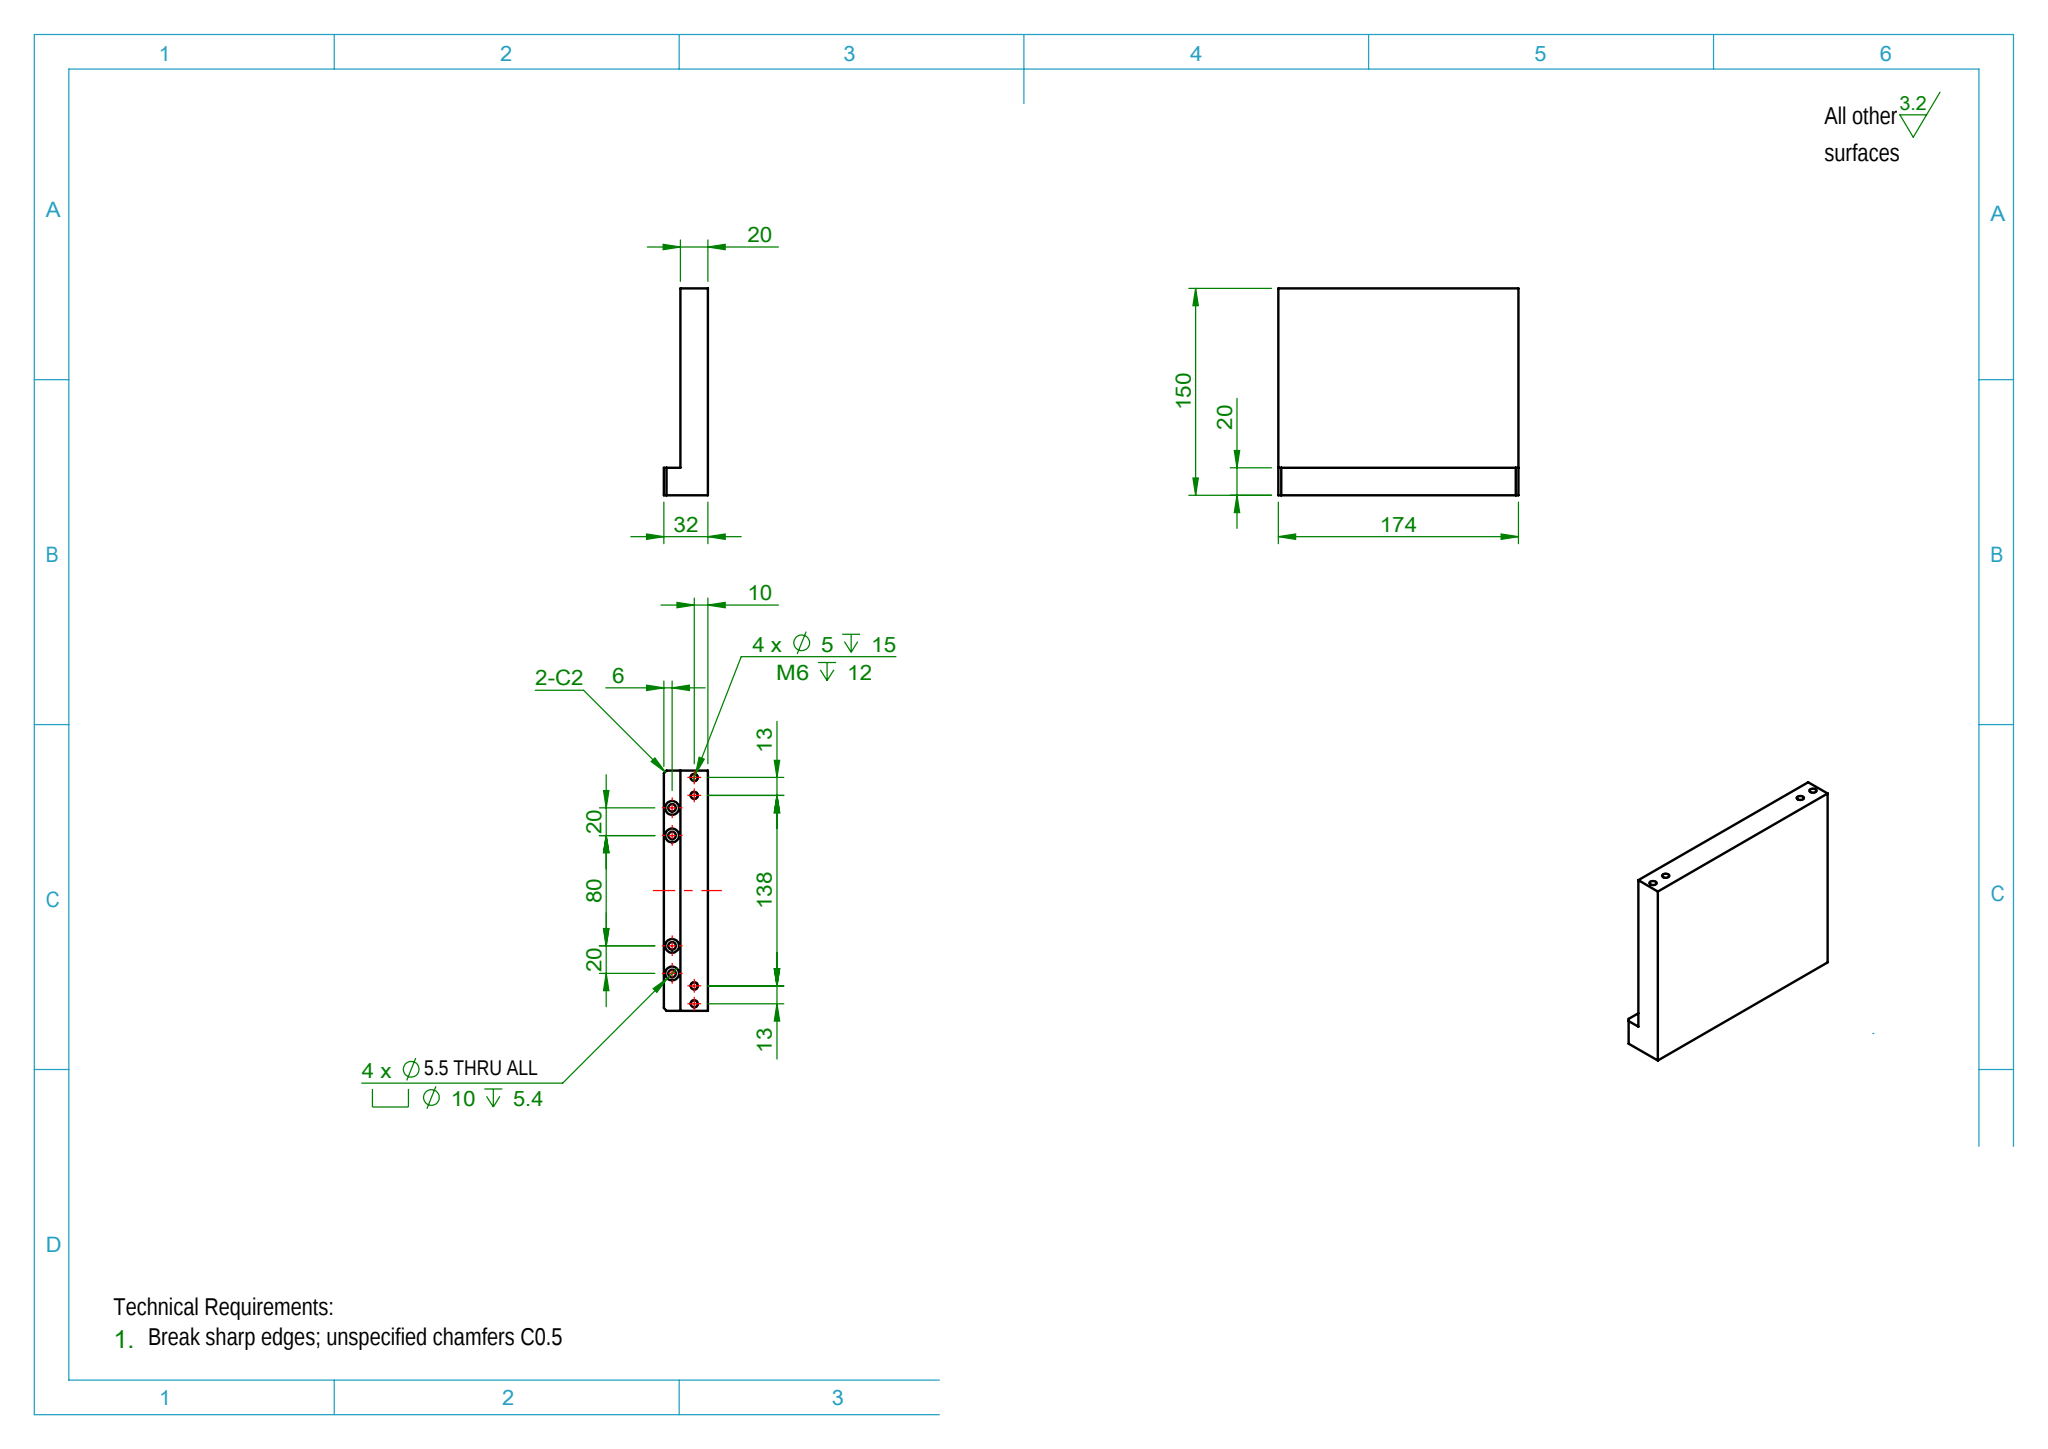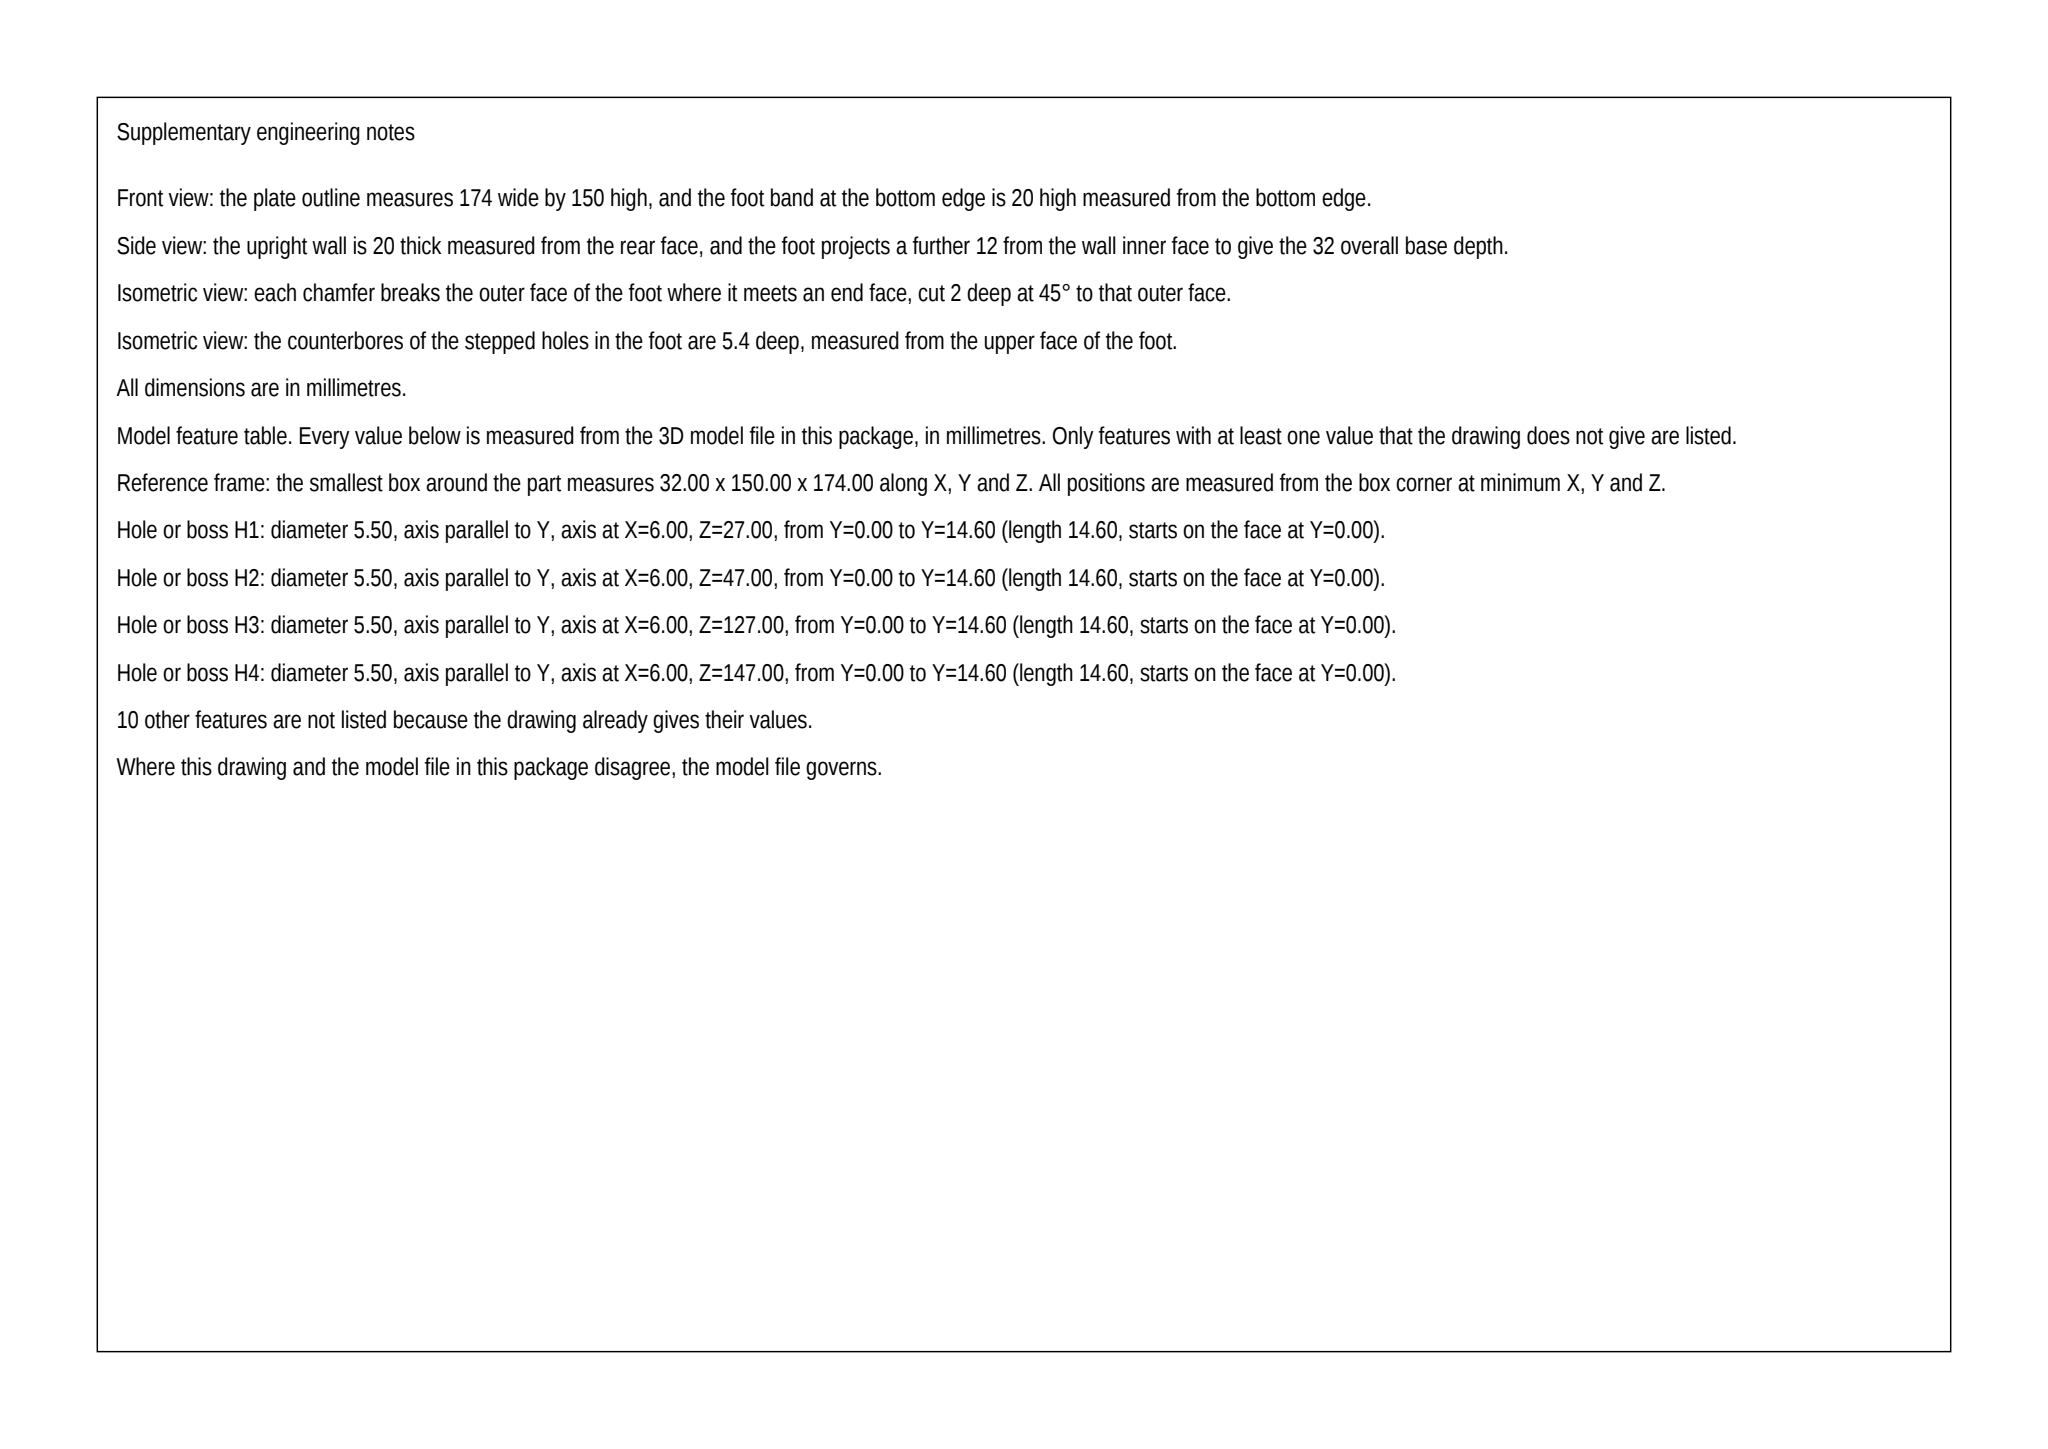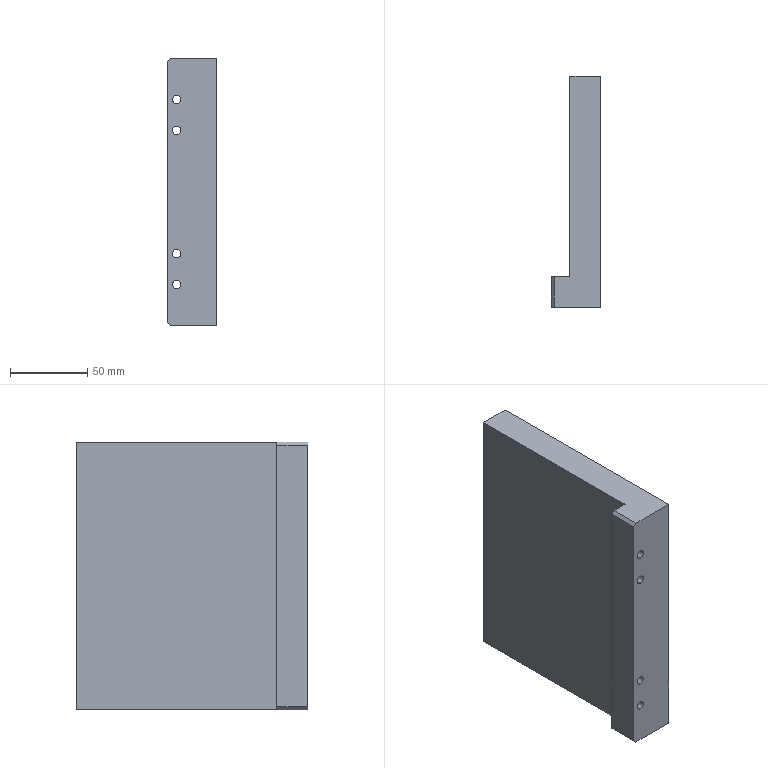Part | SolidWorks | mm | 1 solid | 46 faces | box 32 x 150 x 174 mm | volume 559379 mm3 | cylinder 24 | plane 14 | cone 8 | commonest cylinder face diameters 5 x8 10 x8 5.5 x8
build123d program:
from build123d import *

# Parameters (mm, degrees)
BOSS_EXTRUDE1_DEPTH                             = 174
M5_HEX_SOCKET_HEAD_CAP_SCREW_CBORE1_D           = 5.5
M5_HEX_SOCKET_HEAD_CAP_SCREW_CBORE1_CBORE_D     = 10
M5_HEX_SOCKET_HEAD_CAP_SCREW_CBORE1_CBORE_DEPTH = 5.4
M6_TAPPED_HOLE1_D                               = 5
M6_TAPPED_HOLE1_DEPTH                           = 15
M6_TAPPED_HOLE1_TIP                             = 1.502
CHAMFER1_SIZE                                   = 2


with BuildPart() as part:
    # Sketch1 → Boss-Extrude1 (new body)
    with BuildSketch(Plane.XY):
        Polygon((0, 0), (32, 0), (32, 150), (12, 150), (12, 20), (0, 20), align=None)
    extrude(amount=BOSS_EXTRUDE1_DEPTH)

    # M5 Hex Socket Head Cap Screw CBORE1 (through all)
    with Locations(Plane(origin=(0, 20, 0), x_dir=(1, 0, 0), z_dir=(0, 1, 0))):
        with Locations((6, -147), (6, -127), (6, -47), (6, -27)):
            CounterBoreHole(M5_HEX_SOCKET_HEAD_CAP_SCREW_CBORE1_D / 2, M5_HEX_SOCKET_HEAD_CAP_SCREW_CBORE1_CBORE_D / 2, M5_HEX_SOCKET_HEAD_CAP_SCREW_CBORE1_CBORE_DEPTH)

    # M6 Tapped Hole1
    with Locations(Plane(origin=(0, 150, 0), x_dir=(1, 0, 0), z_dir=(0, 1, 0))):
        with Locations((22, -5), (22, -18), (22, -156), (22, -169)):
            Hole(M6_TAPPED_HOLE1_D / 2, depth=M6_TAPPED_HOLE1_DEPTH)
            with Locations((0, 0, -(M6_TAPPED_HOLE1_DEPTH + M6_TAPPED_HOLE1_TIP / 2))):  # 118° drill point
                Cone(0, M6_TAPPED_HOLE1_D / 2, M6_TAPPED_HOLE1_TIP, mode=Mode.SUBTRACT)

    # Chamfer1
    chamfer1_edges = [part.edges().sort_by_distance(p)[0] for p in [
        (0, 10, 174),
        (0, 10, 0),
    ]]
    chamfer(chamfer1_edges, length=CHAMFER1_SIZE)


solid = part.part